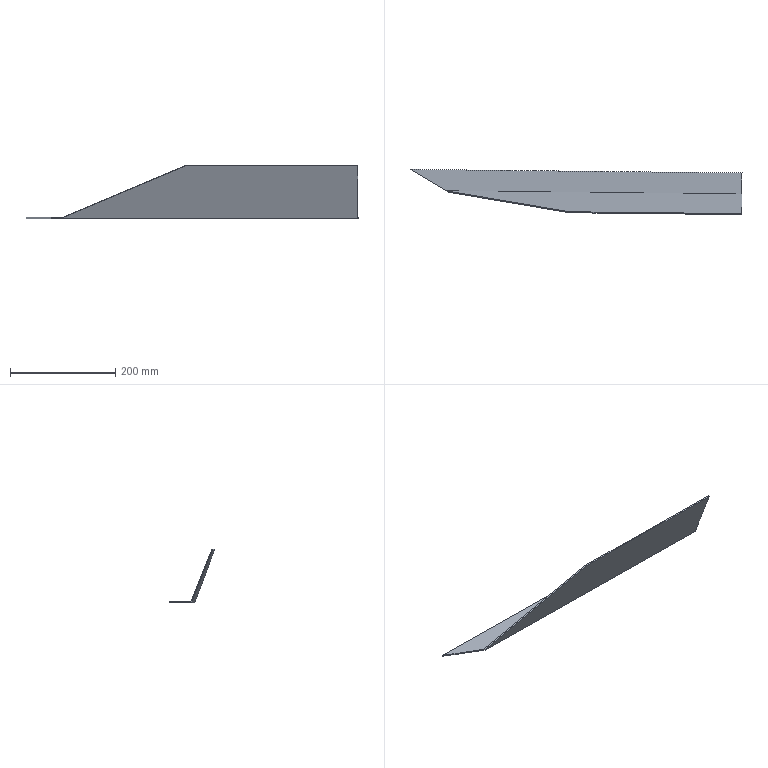Component | SolidWorks | FrontReceivingPlate-1 | 1 solid | 10 faces | box 629.96 x 85.97 x 100.71 mm | volume 142709 mm3 | plane 10
STEP:
#1=COLOUR_RGB('',0.7922,0.8196,0.9333);
#2=FILL_AREA_STYLE_COLOUR('',#1);
#3=FILL_AREA_STYLE('',(#2));
#4=SURFACE_STYLE_FILL_AREA(#3);
#5=SURFACE_SIDE_STYLE('',(#4));
#6=SURFACE_STYLE_USAGE(.BOTH.,#5);
#7=PRESENTATION_STYLE_ASSIGNMENT((#6));
#8=CARTESIAN_POINT('',(18.367,-26.277,-0.5323));
#9=VERTEX_POINT('',#8);
#10=CARTESIAN_POINT('',(18.385,-24.648,-0.5323));
#11=VERTEX_POINT('',#10);
#12=CARTESIAN_POINT('',(18.385,-24.648,-0.5323));
#13=DIRECTION('',(0.0108,0.9999,-0.));
#14=VECTOR('',#13,39.37);
#15=LINE('',#12,#14);
#16=EDGE_CURVE('',#9,#11,#15,.T.);
#17=ORIENTED_EDGE('',*,*,#16,.T.);
#18=CARTESIAN_POINT('',(18.385,-24.648,-0.4535));
#19=VERTEX_POINT('',#18);
#20=CARTESIAN_POINT('',(18.385,-24.648,-0.4535));
#21=DIRECTION('',(0.,-0.,-1.));
#22=VECTOR('',#21,39.37);
#23=LINE('',#20,#22);
#24=EDGE_CURVE('',#19,#11,#23,.T.);
#25=ORIENTED_EDGE('',*,*,#24,.F.);
#26=CARTESIAN_POINT('',(18.368,-26.223,-0.4535));
#27=VERTEX_POINT('',#26);
#28=CARTESIAN_POINT('',(18.385,-24.648,-0.4535));
#29=DIRECTION('',(0.0108,0.9999,-0.));
#30=VECTOR('',#29,39.37);
#31=LINE('',#28,#30);
#32=EDGE_CURVE('',#27,#19,#31,.T.);
#33=ORIENTED_EDGE('',*,*,#32,.F.);
#34=CARTESIAN_POINT('',(18.352,-27.691,3.433));
#35=VERTEX_POINT('',#34);
#36=CARTESIAN_POINT('',(18.368,-26.223,-0.4535));
#37=DIRECTION('',(-0.003816,-0.3535,0.9354));
#38=VECTOR('',#37,39.37);
#39=LINE('',#36,#38);
#40=EDGE_CURVE('',#27,#35,#39,.T.);
#41=ORIENTED_EDGE('',*,*,#40,.T.);
#42=CARTESIAN_POINT('',(18.351,-27.765,3.405));
#43=VERTEX_POINT('',#42);
#44=CARTESIAN_POINT('',(18.352,-27.691,3.433));
#45=DIRECTION('',(-0.0101,-0.9354,-0.3535));
#46=VECTOR('',#45,39.37);
#47=LINE('',#44,#46);
#48=EDGE_CURVE('',#35,#43,#47,.T.);
#49=ORIENTED_EDGE('',*,*,#48,.T.);
#50=CARTESIAN_POINT('',(18.351,-27.765,3.405));
#51=DIRECTION('',(0.003816,0.3535,-0.9354));
#52=VECTOR('',#51,39.37);
#53=LINE('',#50,#52);
#54=EDGE_CURVE('',#43,#9,#53,.T.);
#55=ORIENTED_EDGE('',*,*,#54,.T.);
#56=EDGE_LOOP('',(#17,#25,#33,#41,#49,#55));
#57=FACE_OUTER_BOUND('',#56,.T.);
#58=CARTESIAN_POINT('',(18.385,-24.648,-0.4535));
#59=DIRECTION('',(-0.9999,0.0108,-0.));
#60=DIRECTION('',(-0.,0.,1.));
#61=AXIS2_PLACEMENT_3D('',#58,#59,#60);
#62=PLANE('',#61);
#63=ADVANCED_FACE('',(#57),#62,.F.);
#64=CARTESIAN_POINT('',(-6.417,-24.38,-0.5323));
#65=VERTEX_POINT('',#64);
#66=CARTESIAN_POINT('',(-6.417,-24.38,-0.5323));
#67=DIRECTION('',(-0.9999,0.0108,-0.));
#68=VECTOR('',#67,39.37);
#69=LINE('',#66,#68);
#70=EDGE_CURVE('',#11,#65,#69,.T.);
#71=ORIENTED_EDGE('',*,*,#70,.T.);
#72=CARTESIAN_POINT('',(-6.417,-24.38,-0.4535));
#73=VERTEX_POINT('',#72);
#74=CARTESIAN_POINT('',(-6.417,-24.38,-0.4535));
#75=DIRECTION('',(0.,-0.,-1.));
#76=VECTOR('',#75,39.37);
#77=LINE('',#74,#76);
#78=EDGE_CURVE('',#73,#65,#77,.T.);
#79=ORIENTED_EDGE('',*,*,#78,.F.);
#80=CARTESIAN_POINT('',(-6.417,-24.38,-0.4535));
#81=DIRECTION('',(-0.9999,0.0108,-0.));
#82=VECTOR('',#81,39.37);
#83=LINE('',#80,#82);
#84=EDGE_CURVE('',#19,#73,#83,.T.);
#85=ORIENTED_EDGE('',*,*,#84,.F.);
#86=ORIENTED_EDGE('',*,*,#24,.T.);
#87=EDGE_LOOP('',(#71,#79,#85,#86));
#88=FACE_OUTER_BOUND('',#87,.T.);
#89=CARTESIAN_POINT('',(-6.417,-24.38,-0.4535));
#90=DIRECTION('',(-0.0108,-0.9999,0.));
#91=DIRECTION('',(0.9999,-0.0108,0.));
#92=AXIS2_PLACEMENT_3D('',#89,#90,#91);
#93=PLANE('',#92);
#94=ADVANCED_FACE('',(#88),#93,.F.);
#95=CARTESIAN_POINT('',(-3.706,-25.984,-0.5323));
#96=VERTEX_POINT('',#95);
#97=CARTESIAN_POINT('',(-3.706,-25.984,-0.5323));
#98=DIRECTION('',(0.8606,-0.5093,0.));
#99=VECTOR('',#98,39.37);
#100=LINE('',#97,#99);
#101=EDGE_CURVE('',#65,#96,#100,.T.);
#102=ORIENTED_EDGE('',*,*,#101,.T.);
#103=CARTESIAN_POINT('',(-3.706,-25.984,-0.4535));
#104=VERTEX_POINT('',#103);
#105=CARTESIAN_POINT('',(-3.706,-25.984,-0.4535));
#106=DIRECTION('',(0.,-0.,-1.));
#107=VECTOR('',#106,39.37);
#108=LINE('',#105,#107);
#109=EDGE_CURVE('',#104,#96,#108,.T.);
#110=ORIENTED_EDGE('',*,*,#109,.F.);
#111=CARTESIAN_POINT('',(-3.706,-25.984,-0.4535));
#112=DIRECTION('',(0.8606,-0.5093,0.));
#113=VECTOR('',#112,39.37);
#114=LINE('',#111,#113);
#115=EDGE_CURVE('',#73,#104,#114,.T.);
#116=ORIENTED_EDGE('',*,*,#115,.F.);
#117=ORIENTED_EDGE('',*,*,#78,.T.);
#118=EDGE_LOOP('',(#102,#110,#116,#117));
#119=FACE_OUTER_BOUND('',#118,.T.);
#120=CARTESIAN_POINT('',(-3.706,-25.984,-0.4535));
#121=DIRECTION('',(0.5093,0.8606,0.));
#122=DIRECTION('',(-0.8606,0.5093,-0.));
#123=AXIS2_PLACEMENT_3D('',#120,#121,#122);
#124=PLANE('',#123);
#125=ADVANCED_FACE('',(#119),#124,.F.);
#126=CARTESIAN_POINT('',(18.368,-26.223,-0.4535));
#127=DIRECTION('',(0.9999,-0.0108,0.));
#128=VECTOR('',#127,39.37);
#129=LINE('',#126,#128);
#130=EDGE_CURVE('',#104,#27,#129,.T.);
#131=ORIENTED_EDGE('',*,*,#130,.T.);
#132=ORIENTED_EDGE('',*,*,#32,.T.);
#133=ORIENTED_EDGE('',*,*,#84,.T.);
#134=ORIENTED_EDGE('',*,*,#115,.T.);
#135=EDGE_LOOP('',(#131,#132,#133,#134));
#136=FACE_OUTER_BOUND('',#135,.T.);
#137=CARTESIAN_POINT('',(-1.928,-25.003,-0.4535));
#138=DIRECTION('',(-0.,0.,1.));
#139=DIRECTION('',(0.9999,-0.0108,0.));
#140=AXIS2_PLACEMENT_3D('',#137,#138,#139);
#141=PLANE('',#140);
#142=ADVANCED_FACE('',(#136),#141,.T.);
#143=CARTESIAN_POINT('',(-3.613,-26.04,-0.5323));
#144=VERTEX_POINT('',#143);
#145=CARTESIAN_POINT('',(-3.707,-26.039,-0.5323));
#146=DIRECTION('',(0.9999,-0.0108,0.));
#147=VECTOR('',#146,39.37);
#148=LINE('',#145,#147);
#149=EDGE_CURVE('',#144,#9,#148,.T.);
#150=ORIENTED_EDGE('',*,*,#149,.F.);
#151=CARTESIAN_POINT('',(-3.706,-25.984,-0.5323));
#152=DIRECTION('',(-0.8589,0.5121,-0.));
#153=VECTOR('',#152,39.37);
#154=LINE('',#151,#153);
#155=EDGE_CURVE('',#144,#96,#154,.T.);
#156=ORIENTED_EDGE('',*,*,#155,.T.);
#157=ORIENTED_EDGE('',*,*,#101,.F.);
#158=ORIENTED_EDGE('',*,*,#70,.F.);
#159=ORIENTED_EDGE('',*,*,#16,.F.);
#160=EDGE_LOOP('',(#150,#156,#157,#158,#159));
#161=FACE_OUTER_BOUND('',#160,.T.);
#162=CARTESIAN_POINT('',(-1.928,-25.003,-0.5323));
#163=DIRECTION('',(-0.,0.,1.));
#164=DIRECTION('',(0.9999,-0.0108,0.));
#165=AXIS2_PLACEMENT_3D('',#162,#163,#164);
#166=PLANE('',#165);
#167=ADVANCED_FACE('',(#161),#166,.F.);
#168=CARTESIAN_POINT('',(5.528,-27.626,3.405));
#169=VERTEX_POINT('',#168);
#170=CARTESIAN_POINT('',(-3.533,-26.088,-0.4082));
#171=VERTEX_POINT('',#170);
#172=CARTESIAN_POINT('',(-3.707,-26.058,-0.4813));
#173=DIRECTION('',(-0.9106,0.1546,-0.3832));
#174=VECTOR('',#173,39.37);
#175=LINE('',#172,#174);
#176=EDGE_CURVE('',#169,#171,#175,.T.);
#177=ORIENTED_EDGE('',*,*,#176,.T.);
#178=CARTESIAN_POINT('',(-1.782,-27.131,2.304));
#179=DIRECTION('',(0.5161,-0.3077,0.7994));
#180=VECTOR('',#179,39.37);
#181=LINE('',#178,#180);
#182=EDGE_CURVE('',#144,#171,#181,.T.);
#183=ORIENTED_EDGE('',*,*,#182,.F.);
#184=ORIENTED_EDGE('',*,*,#149,.T.);
#185=ORIENTED_EDGE('',*,*,#54,.F.);
#186=CARTESIAN_POINT('',(-3.723,-27.526,3.405));
#187=DIRECTION('',(0.9999,-0.0108,0.));
#188=VECTOR('',#187,39.37);
#189=LINE('',#186,#188);
#190=EDGE_CURVE('',#169,#43,#189,.T.);
#191=ORIENTED_EDGE('',*,*,#190,.F.);
#192=EDGE_LOOP('',(#177,#183,#184,#185,#191));
#193=FACE_OUTER_BOUND('',#192,.T.);
#194=CARTESIAN_POINT('',(-3.723,-27.526,3.405));
#195=DIRECTION('',(-0.0101,-0.9354,-0.3535));
#196=DIRECTION('',(0.003816,0.3535,-0.9354));
#197=AXIS2_PLACEMENT_3D('',#194,#195,#196);
#198=PLANE('',#197);
#199=ADVANCED_FACE('',(#193),#198,.T.);
#200=CARTESIAN_POINT('',(5.529,-27.553,3.433));
#201=VERTEX_POINT('',#200);
#202=CARTESIAN_POINT('',(5.528,-27.626,3.405));
#203=DIRECTION('',(0.0101,0.9354,0.3535));
#204=VECTOR('',#203,39.37);
#205=LINE('',#202,#204);
#206=EDGE_CURVE('',#169,#201,#205,.T.);
#207=ORIENTED_EDGE('',*,*,#206,.F.);
#208=ORIENTED_EDGE('',*,*,#190,.T.);
#209=ORIENTED_EDGE('',*,*,#48,.F.);
#210=CARTESIAN_POINT('',(-3.722,-27.453,3.433));
#211=DIRECTION('',(0.9999,-0.0108,0.));
#212=VECTOR('',#211,39.37);
#213=LINE('',#210,#212);
#214=EDGE_CURVE('',#201,#35,#213,.T.);
#215=ORIENTED_EDGE('',*,*,#214,.F.);
#216=EDGE_LOOP('',(#207,#208,#209,#215));
#217=FACE_OUTER_BOUND('',#216,.T.);
#218=CARTESIAN_POINT('',(-3.722,-27.453,3.433));
#219=DIRECTION('',(-0.003816,-0.3535,0.9354));
#220=DIRECTION('',(-0.0101,-0.9354,-0.3535));
#221=AXIS2_PLACEMENT_3D('',#218,#219,#220);
#222=PLANE('',#221);
#223=ADVANCED_FACE('',(#217),#222,.T.);
#224=CARTESIAN_POINT('',(-3.706,-25.984,-0.4535));
#225=DIRECTION('',(-0.9106,0.1546,-0.3832));
#226=VECTOR('',#225,39.37);
#227=LINE('',#224,#226);
#228=EDGE_CURVE('',#201,#104,#227,.T.);
#229=ORIENTED_EDGE('',*,*,#228,.F.);
#230=ORIENTED_EDGE('',*,*,#214,.T.);
#231=ORIENTED_EDGE('',*,*,#40,.F.);
#232=ORIENTED_EDGE('',*,*,#130,.F.);
#233=EDGE_LOOP('',(#229,#230,#231,#232));
#234=FACE_OUTER_BOUND('',#233,.T.);
#235=CARTESIAN_POINT('',(-3.706,-25.984,-0.4535));
#236=DIRECTION('',(0.0101,0.9354,0.3535));
#237=DIRECTION('',(-0.003816,-0.3535,0.9354));
#238=AXIS2_PLACEMENT_3D('',#235,#236,#237);
#239=PLANE('',#238);
#240=ADVANCED_FACE('',(#234),#239,.T.);
#241=ORIENTED_EDGE('',*,*,#228,.T.);
#242=CARTESIAN_POINT('',(-3.681,-25.999,-0.4469));
#243=DIRECTION('',(0.838,-0.4996,0.2195));
#244=VECTOR('',#243,39.37);
#245=LINE('',#242,#244);
#246=EDGE_CURVE('',#104,#171,#245,.T.);
#247=ORIENTED_EDGE('',*,*,#246,.T.);
#248=ORIENTED_EDGE('',*,*,#176,.F.);
#249=ORIENTED_EDGE('',*,*,#206,.T.);
#250=EDGE_LOOP('',(#241,#247,#248,#249));
#251=FACE_OUTER_BOUND('',#250,.T.);
#252=CARTESIAN_POINT('',(-3.707,-26.058,-0.4813));
#253=DIRECTION('',(0.4131,0.318,-0.8534));
#254=DIRECTION('',(-0.9015,0.009733,-0.4327));
#255=AXIS2_PLACEMENT_3D('',#252,#253,#254);
#256=PLANE('',#255);
#257=ADVANCED_FACE('',(#251),#256,.F.);
#258=ORIENTED_EDGE('',*,*,#182,.T.);
#259=ORIENTED_EDGE('',*,*,#246,.F.);
#260=ORIENTED_EDGE('',*,*,#109,.T.);
#261=ORIENTED_EDGE('',*,*,#155,.F.);
#262=EDGE_LOOP('',(#258,#259,#260,#261));
#263=FACE_OUTER_BOUND('',#262,.T.);
#264=CARTESIAN_POINT('',(-3.706,-25.984,-0.5323));
#265=DIRECTION('',(0.5121,0.8589,0.));
#266=DIRECTION('',(-0.8589,0.5121,-0.));
#267=AXIS2_PLACEMENT_3D('',#264,#265,#266);
#268=PLANE('',#267);
#269=ADVANCED_FACE('',(#263),#268,.F.);
#270=CLOSED_SHELL('',(#63,#94,#125,#142,#167,#199,#223,#240,#257,#269));
#271=MANIFOLD_SOLID_BREP('',#270);
#272=STYLED_ITEM('',(#7),#271);
#273=(LENGTH_UNIT()NAMED_UNIT(*)SI_UNIT($,.METRE.));
#274=LENGTH_MEASURE_WITH_UNIT(LENGTH_MEASURE(0.0254),#273);
#275=DIMENSIONAL_EXPONENTS(1.,0.,0.,0.,0.,0.,0.);
#276=(CONVERSION_BASED_UNIT('',#274)LENGTH_UNIT()NAMED_UNIT(#275));
#277=UNCERTAINTY_MEASURE_WITH_UNIT(LENGTH_MEASURE(0.00001),#276,'','');
#278=(NAMED_UNIT(*)PLANE_ANGLE_UNIT()SI_UNIT($,.RADIAN.));
#279=(NAMED_UNIT(*)SI_UNIT($,.STERADIAN.)SOLID_ANGLE_UNIT());
#280=(GEOMETRIC_REPRESENTATION_CONTEXT(3)GLOBAL_UNCERTAINTY_ASSIGNED_CONTEXT((#277))GLOBAL_UNIT_ASSIGNED_CONTEXT((#276,#278,#279))REPRESENTATION_CONTEXT('',''));
#281=MECHANICAL_DESIGN_GEOMETRIC_PRESENTATION_REPRESENTATION('',(#272),#280);
#282=PRESENTATION_LAYER_ASSIGNMENT('','',(#272));
#283=CARTESIAN_POINT('',(0.,0.,0.));
#284=DIRECTION('',(0.,0.,1.));
#285=DIRECTION('',(1.,0.,0.));
#286=AXIS2_PLACEMENT_3D('',#283,#284,#285);
#287=(LENGTH_UNIT()NAMED_UNIT(*)SI_UNIT($,.METRE.));
#288=LENGTH_MEASURE_WITH_UNIT(LENGTH_MEASURE(0.0254),#287);
#289=DIMENSIONAL_EXPONENTS(1.,0.,0.,0.,0.,0.,0.);
#290=(CONVERSION_BASED_UNIT('',#288)LENGTH_UNIT()NAMED_UNIT(#289));
#291=UNCERTAINTY_MEASURE_WITH_UNIT(LENGTH_MEASURE(0.00001),#290,'','');
#292=(NAMED_UNIT(*)PLANE_ANGLE_UNIT()SI_UNIT($,.RADIAN.));
#293=(NAMED_UNIT(*)SI_UNIT($,.STERADIAN.)SOLID_ANGLE_UNIT());
#294=(GEOMETRIC_REPRESENTATION_CONTEXT(3)GLOBAL_UNCERTAINTY_ASSIGNED_CONTEXT((#291))GLOBAL_UNIT_ASSIGNED_CONTEXT((#290,#292,#293))REPRESENTATION_CONTEXT('',''));
#295=ADVANCED_BREP_SHAPE_REPRESENTATION('',(#271,#286),#294);